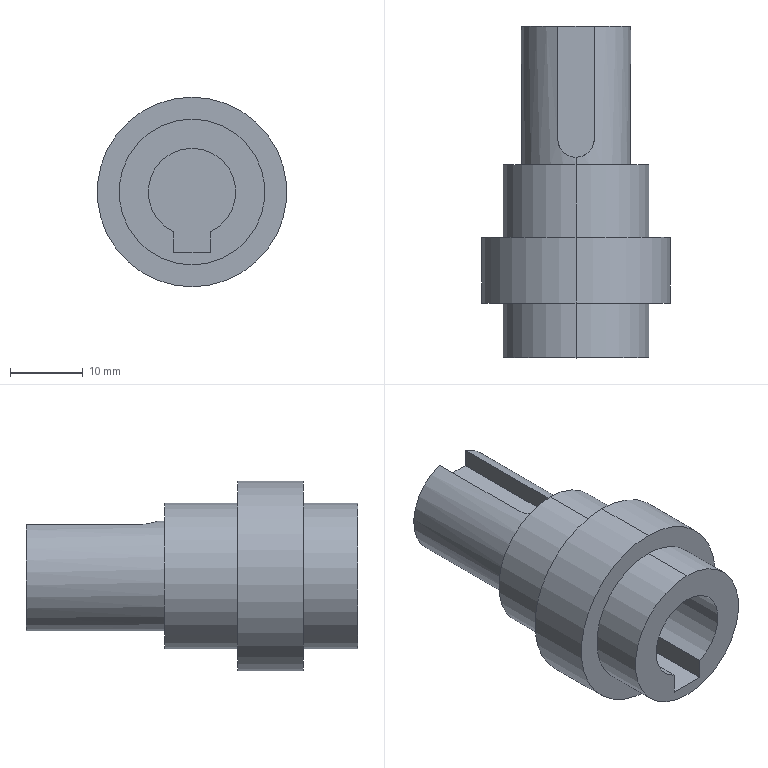Component | SolidWorks | DialAxis-1_DialAxisNo.3-1 | 1 solid | 26 faces | box 26 x 45.5 x 26 mm | volume 10013 mm3 | cylinder 12 | plane 12 | cone 2 | commonest cylinder face diameters 20 x4 3 x2 26 x2 15 x2 5 x1 12 x1
build123d program:
from build123d import *

# Parameters (mm, degrees)
CUT_EXTRUDE1_DEPTH    = 10
SKETCH3_R             = 6
CUT_EXTRUDE2_DEPTH    = 26
CUT_EXTRUDE3_DEPTH    = 26
M3_TAPPED_HOLE1_D     = 3
M3_TAPPED_HOLE1_DEPTH = 15
M3_TAPPED_HOLE1_TIP   = 0.9013


with BuildPart() as part:
    # Sketch1 → Revolve1 (revolve)
    with BuildSketch(Plane.XY, mode=Mode.PRIVATE) as revolve1_sk:
        Polygon((-29, 0), (-29, 7.5), (-10, 7.5), (-10, 10), (0, 10), (0, 13), (9, 13), (9, 10), (16.5, 10), (16.5, 9), (16.5, 0), align=None)
    revolve(revolve1_sk.sketch.rotate(Axis((-29, 0, 0), (1, 0, 0)), 90), axis=Axis((-29, 0, 0), (1, 0, 0)))

    # Sketch2 → Cut-Extrude1 (cut)
    with BuildSketch(Plane.XY.offset(4.5)):
        with BuildLine():
            Line((-29, 2.5), (-13.5, 2.5))
            ThreePointArc((-13.5, 2.5), (-11, 0), (-13.5, -2.5))
            Line((-13.5, -2.5), (-29, -2.5))
            ThreePointArc((-29, -2.5), (-31.5, 0), (-29, 2.5))
        make_face()
    extrude(amount=CUT_EXTRUDE1_DEPTH, mode=Mode.SUBTRACT)

    # Sketch3 → Cut-Extrude2 (cut)
    with BuildSketch(Plane(origin=(16.5, 0, 0), x_dir=(0, 0, -1), z_dir=(1, 0, 0))):
        Circle(SKETCH3_R)
    extrude(amount=-CUT_EXTRUDE2_DEPTH, mode=Mode.SUBTRACT)

    # Sketch4 → Cut-Extrude3 (cut)
    with BuildSketch(Plane(origin=(16.5, 0, 0), x_dir=(0, 0, -1), z_dir=(1, 0, 0))):
        with BuildLine():
            Line((8.3, 0), (6, 0))
            ThreePointArc((6, 0), (5.862, -1.279), (5.454, -2.5))
            Line((5.454, -2.5), (8.3, -2.5))
            Line((8.3, -2.5), (8.3, 0))
        make_face()
        with BuildLine():
            ThreePointArc((5.454, 2.5), (5.862, 1.279), (6, 0))
            Line((6, 0), (8.3, 0))
            Line((8.3, 0), (8.3, 2.5))
            Line((8.3, 2.5), (5.454, 2.5))
        make_face()
    extrude(amount=-CUT_EXTRUDE3_DEPTH, mode=Mode.SUBTRACT)

    # M3 Tapped Hole1
    with Locations(Plane.ZY.offset(29)):
        with Locations((0, 0)):
            Hole(M3_TAPPED_HOLE1_D / 2, depth=M3_TAPPED_HOLE1_DEPTH)
            with Locations((0, 0, -(M3_TAPPED_HOLE1_DEPTH + M3_TAPPED_HOLE1_TIP / 2))):  # 118° drill point
                Cone(0, M3_TAPPED_HOLE1_D / 2, M3_TAPPED_HOLE1_TIP, mode=Mode.SUBTRACT)


solid = part.part

# Placed as in the assembly
solid = solid.moved(Location((-96.534, 127.266, -166.507), (0, 0, -90)))
STEP:
#1=COLOUR_RGB('',0.7922,0.8196,0.9333);
#2=FILL_AREA_STYLE_COLOUR('',#1);
#3=FILL_AREA_STYLE('',(#2));
#4=SURFACE_STYLE_FILL_AREA(#3);
#5=SURFACE_SIDE_STYLE('',(#4));
#6=SURFACE_STYLE_USAGE(.BOTH.,#5);
#7=PRESENTATION_STYLE_ASSIGNMENT((#6));
#8=CARTESIAN_POINT('',(-3.801,5.562,-6.614));
#9=VERTEX_POINT('',#8);
#10=CARTESIAN_POINT('',(-3.801,5.562,-6.496));
#11=VERTEX_POINT('',#10);
#12=CARTESIAN_POINT('',(-3.801,5.562,-6.555));
#13=DIRECTION('',(0.,1.,0.));
#14=DIRECTION('',(0.,0.,1.));
#15=AXIS2_PLACEMENT_3D('',#12,#13,#14);
#16=CIRCLE('',#15,0.05906);
#17=EDGE_CURVE('',#9,#11,#16,.T.);
#18=ORIENTED_EDGE('',*,*,#17,.F.);
#19=CARTESIAN_POINT('',(-3.801,6.152,-6.614));
#20=VERTEX_POINT('',#19);
#21=CARTESIAN_POINT('',(-3.801,6.152,-6.614));
#22=DIRECTION('',(0.,1.,0.));
#23=VECTOR('',#22,39.37);
#24=LINE('',#21,#23);
#25=EDGE_CURVE('',#9,#20,#24,.T.);
#26=ORIENTED_EDGE('',*,*,#25,.T.);
#27=CARTESIAN_POINT('',(-3.801,6.152,-6.496));
#28=VERTEX_POINT('',#27);
#29=CARTESIAN_POINT('',(-3.801,6.152,-6.555));
#30=DIRECTION('',(0.,1.,0.));
#31=DIRECTION('',(0.,0.,1.));
#32=AXIS2_PLACEMENT_3D('',#29,#30,#31);
#33=CIRCLE('',#32,0.05906);
#34=EDGE_CURVE('',#20,#28,#33,.T.);
#35=ORIENTED_EDGE('',*,*,#34,.T.);
#36=CARTESIAN_POINT('',(-3.801,6.152,-6.496));
#37=DIRECTION('',(0.,1.,0.));
#38=VECTOR('',#37,39.37);
#39=LINE('',#36,#38);
#40=EDGE_CURVE('',#11,#28,#39,.T.);
#41=ORIENTED_EDGE('',*,*,#40,.F.);
#42=EDGE_LOOP('',(#18,#26,#35,#41));
#43=FACE_OUTER_BOUND('',#42,.T.);
#44=CARTESIAN_POINT('',(-3.801,6.152,-6.555));
#45=DIRECTION('',(0.,1.,0.));
#46=DIRECTION('',(0.,0.,1.));
#47=AXIS2_PLACEMENT_3D('',#44,#45,#46);
#48=CYLINDRICAL_SURFACE('',#47,0.05906);
#49=ADVANCED_FACE('',(#43),#48,.F.);
#50=CARTESIAN_POINT('',(-3.801,5.526,-6.555));
#51=VERTEX_POINT('',#50);
#52=CARTESIAN_POINT('',(-3.801,5.562,-6.496));
#53=DIRECTION('',(0.,0.515,0.8572));
#54=VECTOR('',#53,39.37);
#55=LINE('',#52,#54);
#56=EDGE_CURVE('',#51,#11,#55,.T.);
#57=ORIENTED_EDGE('',*,*,#56,.F.);
#58=CARTESIAN_POINT('',(-3.801,5.562,-6.614));
#59=DIRECTION('',(-0.,0.515,-0.8572));
#60=VECTOR('',#59,39.37);
#61=LINE('',#58,#60);
#62=EDGE_CURVE('',#51,#9,#61,.T.);
#63=ORIENTED_EDGE('',*,*,#62,.T.);
#64=ORIENTED_EDGE('',*,*,#17,.T.);
#65=EDGE_LOOP('',(#57,#63,#64));
#66=FACE_OUTER_BOUND('',#65,.T.);
#67=CARTESIAN_POINT('',(-3.801,5.562,-6.555));
#68=DIRECTION('',(0.,1.,0.));
#69=DIRECTION('',(0.,0.,1.));
#70=AXIS2_PLACEMENT_3D('',#67,#68,#69);
#71=CONICAL_SURFACE('',#70,0.05906,1.03);
#72=ADVANCED_FACE('',(#66),#71,.F.);
#73=CARTESIAN_POINT('',(-3.801,4.361,-6.162));
#74=VERTEX_POINT('',#73);
#75=CARTESIAN_POINT('',(-3.801,4.361,-6.949));
#76=VERTEX_POINT('',#75);
#77=CARTESIAN_POINT('',(-3.801,4.361,-6.555));
#78=DIRECTION('',(0.,1.,0.));
#79=DIRECTION('',(0.,0.,1.));
#80=AXIS2_PLACEMENT_3D('',#77,#78,#79);
#81=CIRCLE('',#80,0.3937);
#82=EDGE_CURVE('',#74,#76,#81,.T.);
#83=ORIENTED_EDGE('',*,*,#82,.T.);
#84=CARTESIAN_POINT('',(-3.801,4.656,-6.949));
#85=VERTEX_POINT('',#84);
#86=CARTESIAN_POINT('',(-3.801,6.152,-6.949));
#87=DIRECTION('',(0.,1.,0.));
#88=VECTOR('',#87,39.37);
#89=LINE('',#86,#88);
#90=EDGE_CURVE('',#76,#85,#89,.T.);
#91=ORIENTED_EDGE('',*,*,#90,.T.);
#92=CARTESIAN_POINT('',(-3.801,4.656,-6.162));
#93=VERTEX_POINT('',#92);
#94=CARTESIAN_POINT('',(-3.801,4.656,-6.555));
#95=DIRECTION('',(0.,1.,0.));
#96=DIRECTION('',(0.,0.,1.));
#97=AXIS2_PLACEMENT_3D('',#94,#95,#96);
#98=CIRCLE('',#97,0.3937);
#99=EDGE_CURVE('',#93,#85,#98,.T.);
#100=ORIENTED_EDGE('',*,*,#99,.F.);
#101=CARTESIAN_POINT('',(-3.801,6.152,-6.162));
#102=DIRECTION('',(0.,1.,0.));
#103=VECTOR('',#102,39.37);
#104=LINE('',#101,#103);
#105=EDGE_CURVE('',#74,#93,#104,.T.);
#106=ORIENTED_EDGE('',*,*,#105,.F.);
#107=EDGE_LOOP('',(#83,#91,#100,#106));
#108=FACE_OUTER_BOUND('',#107,.T.);
#109=CARTESIAN_POINT('',(-3.801,6.152,-6.555));
#110=DIRECTION('',(0.,1.,0.));
#111=DIRECTION('',(0.,0.,1.));
#112=AXIS2_PLACEMENT_3D('',#109,#110,#111);
#113=CYLINDRICAL_SURFACE('',#112,0.3937);
#114=ADVANCED_FACE('',(#108),#113,.T.);
#115=CARTESIAN_POINT('',(-3.801,4.656,-6.044));
#116=VERTEX_POINT('',#115);
#117=CARTESIAN_POINT('',(-3.801,4.656,-7.067));
#118=VERTEX_POINT('',#117);
#119=CARTESIAN_POINT('',(-3.801,4.656,-6.555));
#120=DIRECTION('',(0.,1.,0.));
#121=DIRECTION('',(0.,0.,1.));
#122=AXIS2_PLACEMENT_3D('',#119,#120,#121);
#123=CIRCLE('',#122,0.5118);
#124=EDGE_CURVE('',#116,#118,#123,.T.);
#125=ORIENTED_EDGE('',*,*,#124,.T.);
#126=CARTESIAN_POINT('',(-3.801,5.01,-7.067));
#127=VERTEX_POINT('',#126);
#128=CARTESIAN_POINT('',(-3.801,6.152,-7.067));
#129=DIRECTION('',(0.,1.,0.));
#130=VECTOR('',#129,39.37);
#131=LINE('',#128,#130);
#132=EDGE_CURVE('',#118,#127,#131,.T.);
#133=ORIENTED_EDGE('',*,*,#132,.T.);
#134=CARTESIAN_POINT('',(-3.801,5.01,-6.044));
#135=VERTEX_POINT('',#134);
#136=CARTESIAN_POINT('',(-3.801,5.01,-6.555));
#137=DIRECTION('',(0.,1.,0.));
#138=DIRECTION('',(0.,0.,1.));
#139=AXIS2_PLACEMENT_3D('',#136,#137,#138);
#140=CIRCLE('',#139,0.5118);
#141=EDGE_CURVE('',#135,#127,#140,.T.);
#142=ORIENTED_EDGE('',*,*,#141,.F.);
#143=CARTESIAN_POINT('',(-3.801,6.152,-6.044));
#144=DIRECTION('',(0.,1.,0.));
#145=VECTOR('',#144,39.37);
#146=LINE('',#143,#145);
#147=EDGE_CURVE('',#116,#135,#146,.T.);
#148=ORIENTED_EDGE('',*,*,#147,.F.);
#149=EDGE_LOOP('',(#125,#133,#142,#148));
#150=FACE_OUTER_BOUND('',#149,.T.);
#151=CARTESIAN_POINT('',(-3.801,6.152,-6.555));
#152=DIRECTION('',(0.,1.,0.));
#153=DIRECTION('',(0.,0.,1.));
#154=AXIS2_PLACEMENT_3D('',#151,#152,#153);
#155=CYLINDRICAL_SURFACE('',#154,0.5118);
#156=ADVANCED_FACE('',(#150),#155,.T.);
#157=CARTESIAN_POINT('',(-3.801,5.01,-6.162));
#158=VERTEX_POINT('',#157);
#159=CARTESIAN_POINT('',(-3.801,5.01,-6.949));
#160=VERTEX_POINT('',#159);
#161=CARTESIAN_POINT('',(-3.801,5.01,-6.555));
#162=DIRECTION('',(0.,1.,0.));
#163=DIRECTION('',(0.,0.,1.));
#164=AXIS2_PLACEMENT_3D('',#161,#162,#163);
#165=CIRCLE('',#164,0.3937);
#166=EDGE_CURVE('',#158,#160,#165,.T.);
#167=ORIENTED_EDGE('',*,*,#166,.T.);
#168=CARTESIAN_POINT('',(-3.801,5.404,-6.949));
#169=VERTEX_POINT('',#168);
#170=CARTESIAN_POINT('',(-3.801,6.152,-6.949));
#171=DIRECTION('',(0.,1.,0.));
#172=VECTOR('',#171,39.37);
#173=LINE('',#170,#172);
#174=EDGE_CURVE('',#160,#169,#173,.T.);
#175=ORIENTED_EDGE('',*,*,#174,.T.);
#176=CARTESIAN_POINT('',(-3.801,5.404,-6.162));
#177=VERTEX_POINT('',#176);
#178=CARTESIAN_POINT('',(-3.801,5.404,-6.555));
#179=DIRECTION('',(0.,1.,0.));
#180=DIRECTION('',(0.,0.,1.));
#181=AXIS2_PLACEMENT_3D('',#178,#179,#180);
#182=CIRCLE('',#181,0.3937);
#183=EDGE_CURVE('',#177,#169,#182,.T.);
#184=ORIENTED_EDGE('',*,*,#183,.F.);
#185=CARTESIAN_POINT('',(-3.801,6.152,-6.162));
#186=DIRECTION('',(0.,1.,0.));
#187=VECTOR('',#186,39.37);
#188=LINE('',#185,#187);
#189=EDGE_CURVE('',#158,#177,#188,.T.);
#190=ORIENTED_EDGE('',*,*,#189,.F.);
#191=EDGE_LOOP('',(#167,#175,#184,#190));
#192=FACE_OUTER_BOUND('',#191,.T.);
#193=CARTESIAN_POINT('',(-3.801,6.152,-6.555));
#194=DIRECTION('',(0.,1.,0.));
#195=DIRECTION('',(0.,0.,1.));
#196=AXIS2_PLACEMENT_3D('',#193,#194,#195);
#197=CYLINDRICAL_SURFACE('',#196,0.3937);
#198=ADVANCED_FACE('',(#192),#197,.T.);
#199=CARTESIAN_POINT('',(-3.801,5.404,-6.26));
#200=VERTEX_POINT('',#199);
#201=CARTESIAN_POINT('',(-3.801,5.404,-6.851));
#202=VERTEX_POINT('',#201);
#203=CARTESIAN_POINT('',(-3.801,5.404,-6.555));
#204=DIRECTION('',(0.,1.,0.));
#205=DIRECTION('',(0.,0.,1.));
#206=AXIS2_PLACEMENT_3D('',#203,#204,#205);
#207=CIRCLE('',#206,0.2953);
#208=EDGE_CURVE('',#200,#202,#207,.T.);
#209=ORIENTED_EDGE('',*,*,#208,.T.);
#210=CARTESIAN_POINT('',(-3.801,6.152,-6.851));
#211=VERTEX_POINT('',#210);
#212=CARTESIAN_POINT('',(-3.801,6.152,-6.851));
#213=DIRECTION('',(0.,1.,0.));
#214=VECTOR('',#213,39.37);
#215=LINE('',#212,#214);
#216=EDGE_CURVE('',#202,#211,#215,.T.);
#217=ORIENTED_EDGE('',*,*,#216,.T.);
#218=CARTESIAN_POINT('',(-3.702,6.152,-6.277));
#219=VERTEX_POINT('',#218);
#220=CARTESIAN_POINT('',(-3.801,6.152,-6.555));
#221=DIRECTION('',(0.,1.,0.));
#222=DIRECTION('',(0.,0.,1.));
#223=AXIS2_PLACEMENT_3D('',#220,#221,#222);
#224=CIRCLE('',#223,0.2953);
#225=EDGE_CURVE('',#219,#211,#224,.T.);
#226=ORIENTED_EDGE('',*,*,#225,.F.);
#227=CARTESIAN_POINT('',(-3.702,5.542,-6.277));
#228=VERTEX_POINT('',#227);
#229=CARTESIAN_POINT('',(-3.702,6.152,-6.277));
#230=DIRECTION('',(0.,1.,0.));
#231=VECTOR('',#230,39.37);
#232=LINE('',#229,#231);
#233=EDGE_CURVE('',#228,#219,#232,.T.);
#234=ORIENTED_EDGE('',*,*,#233,.F.);
#235=CARTESIAN_POINT('',(-3.801,5.444,-6.26));
#236=VERTEX_POINT('',#235);
#237=CARTESIAN_POINT('',(-3.801,5.444,-6.26));
#238=CARTESIAN_POINT('',(-3.794,5.444,-6.26));
#239=CARTESIAN_POINT('',(-3.788,5.444,-6.26));
#240=CARTESIAN_POINT('',(-3.775,5.447,-6.261));
#241=CARTESIAN_POINT('',(-3.769,5.449,-6.262));
#242=CARTESIAN_POINT('',(-3.757,5.454,-6.263));
#243=CARTESIAN_POINT('',(-3.751,5.457,-6.264));
#244=CARTESIAN_POINT('',(-3.74,5.464,-6.266));
#245=CARTESIAN_POINT('',(-3.735,5.468,-6.267));
#246=CARTESIAN_POINT('',(-3.726,5.477,-6.27));
#247=CARTESIAN_POINT('',(-3.722,5.482,-6.271));
#248=CARTESIAN_POINT('',(-3.715,5.492,-6.273));
#249=CARTESIAN_POINT('',(-3.712,5.498,-6.274));
#250=CARTESIAN_POINT('',(-3.707,5.51,-6.275));
#251=CARTESIAN_POINT('',(-3.705,5.516,-6.276));
#252=CARTESIAN_POINT('',(-3.703,5.529,-6.277));
#253=CARTESIAN_POINT('',(-3.702,5.535,-6.277));
#254=CARTESIAN_POINT('',(-3.702,5.542,-6.277));
#255=B_SPLINE_CURVE_WITH_KNOTS('',3,(#237,#238,#239,#240,#241,#242,#243,#244,#245,#246,#247,#248,#249,#250,#251,#252,#253,#254),.UNSPECIFIED.,.F.,.F.,(4,2,2,2,2,2,2,2,4),(0.003937,0.004429,0.004921,0.005412,0.005904,0.006395,0.006887,0.007378,0.00787),.UNSPECIFIED.);
#256=EDGE_CURVE('',#236,#228,#255,.T.);
#257=ORIENTED_EDGE('',*,*,#256,.F.);
#258=CARTESIAN_POINT('',(-3.801,6.152,-6.26));
#259=DIRECTION('',(0.,1.,0.));
#260=VECTOR('',#259,39.37);
#261=LINE('',#258,#260);
#262=EDGE_CURVE('',#200,#236,#261,.T.);
#263=ORIENTED_EDGE('',*,*,#262,.F.);
#264=EDGE_LOOP('',(#209,#217,#226,#234,#257,#263));
#265=FACE_OUTER_BOUND('',#264,.T.);
#266=CARTESIAN_POINT('',(-3.801,6.152,-6.555));
#267=DIRECTION('',(0.,1.,0.));
#268=DIRECTION('',(0.,0.,1.));
#269=AXIS2_PLACEMENT_3D('',#266,#267,#268);
#270=CYLINDRICAL_SURFACE('',#269,0.2953);
#271=ADVANCED_FACE('',(#265),#270,.T.);
#272=CARTESIAN_POINT('',(-3.801,6.152,-6.555));
#273=DIRECTION('',(0.,1.,0.));
#274=DIRECTION('',(0.,0.,1.));
#275=AXIS2_PLACEMENT_3D('',#272,#273,#274);
#276=CIRCLE('',#275,0.05906);
#277=EDGE_CURVE('',#28,#20,#276,.T.);
#278=ORIENTED_EDGE('',*,*,#277,.F.);
#279=ORIENTED_EDGE('',*,*,#34,.F.);
#280=EDGE_LOOP('',(#278,#279));
#281=FACE_BOUND('',#280,.T.);
#282=CARTESIAN_POINT('',(-3.899,6.152,-6.277));
#283=VERTEX_POINT('',#282);
#284=CARTESIAN_POINT('',(-3.899,6.152,-6.378));
#285=VERTEX_POINT('',#284);
#286=CARTESIAN_POINT('',(-3.899,6.152,-5.985));
#287=DIRECTION('',(-0.,0.,-1.));
#288=VECTOR('',#287,39.37);
#289=LINE('',#286,#288);
#290=EDGE_CURVE('',#283,#285,#289,.T.);
#291=ORIENTED_EDGE('',*,*,#290,.T.);
#292=CARTESIAN_POINT('',(-3.702,6.152,-6.378));
#293=VERTEX_POINT('',#292);
#294=CARTESIAN_POINT('',(-3.801,6.152,-6.378));
#295=DIRECTION('',(-1.,0.,0.));
#296=VECTOR('',#295,39.37);
#297=LINE('',#294,#296);
#298=EDGE_CURVE('',#293,#285,#297,.T.);
#299=ORIENTED_EDGE('',*,*,#298,.F.);
#300=CARTESIAN_POINT('',(-3.702,6.152,-5.985));
#301=DIRECTION('',(-0.,0.,-1.));
#302=VECTOR('',#301,39.37);
#303=LINE('',#300,#302);
#304=EDGE_CURVE('',#219,#293,#303,.T.);
#305=ORIENTED_EDGE('',*,*,#304,.F.);
#306=ORIENTED_EDGE('',*,*,#225,.T.);
#307=CARTESIAN_POINT('',(-3.801,6.152,-6.555));
#308=DIRECTION('',(0.,1.,0.));
#309=DIRECTION('',(0.,0.,1.));
#310=AXIS2_PLACEMENT_3D('',#307,#308,#309);
#311=CIRCLE('',#310,0.2953);
#312=EDGE_CURVE('',#211,#283,#311,.T.);
#313=ORIENTED_EDGE('',*,*,#312,.T.);
#314=EDGE_LOOP('',(#291,#299,#305,#306,#313));
#315=FACE_OUTER_BOUND('',#314,.T.);
#316=CARTESIAN_POINT('',(-3.801,6.152,-6.555));
#317=DIRECTION('',(0.,-1.,0.));
#318=DIRECTION('',(-0.,0.,-1.));
#319=AXIS2_PLACEMENT_3D('',#316,#317,#318);
#320=PLANE('',#319);
#321=ADVANCED_FACE('',(#281,#315),#320,.F.);
#322=ORIENTED_EDGE('',*,*,#216,.F.);
#323=CARTESIAN_POINT('',(-3.801,5.404,-6.555));
#324=DIRECTION('',(0.,1.,0.));
#325=DIRECTION('',(0.,0.,1.));
#326=AXIS2_PLACEMENT_3D('',#323,#324,#325);
#327=CIRCLE('',#326,0.2953);
#328=EDGE_CURVE('',#202,#200,#327,.T.);
#329=ORIENTED_EDGE('',*,*,#328,.T.);
#330=ORIENTED_EDGE('',*,*,#262,.T.);
#331=CARTESIAN_POINT('',(-3.899,5.542,-6.277));
#332=VERTEX_POINT('',#331);
#333=CARTESIAN_POINT('',(-3.899,5.542,-6.277));
#334=CARTESIAN_POINT('',(-3.899,5.535,-6.277));
#335=CARTESIAN_POINT('',(-3.898,5.529,-6.277));
#336=CARTESIAN_POINT('',(-3.896,5.516,-6.276));
#337=CARTESIAN_POINT('',(-3.894,5.51,-6.275));
#338=CARTESIAN_POINT('',(-3.889,5.498,-6.274));
#339=CARTESIAN_POINT('',(-3.886,5.493,-6.273));
#340=CARTESIAN_POINT('',(-3.879,5.482,-6.271));
#341=CARTESIAN_POINT('',(-3.875,5.477,-6.27));
#342=CARTESIAN_POINT('',(-3.861,5.463,-6.266));
#343=CARTESIAN_POINT('',(-3.85,5.456,-6.264));
#344=CARTESIAN_POINT('',(-3.832,5.449,-6.262));
#345=CARTESIAN_POINT('',(-3.826,5.447,-6.261));
#346=CARTESIAN_POINT('',(-3.813,5.444,-6.26));
#347=CARTESIAN_POINT('',(-3.807,5.444,-6.26));
#348=CARTESIAN_POINT('',(-3.801,5.444,-6.26));
#349=B_SPLINE_CURVE_WITH_KNOTS('',3,(#333,#334,#335,#336,#337,#338,#339,#340,#341,#342,#343,#344,#345,#346,#347,#348),.UNSPECIFIED.,.F.,.F.,(4,2,2,2,2,2,2,4),(0.,0.0004922,0.0009844,0.001477,0.001969,0.002953,0.003445,0.003937),.UNSPECIFIED.);
#350=EDGE_CURVE('',#332,#236,#349,.T.);
#351=ORIENTED_EDGE('',*,*,#350,.F.);
#352=CARTESIAN_POINT('',(-3.899,6.152,-6.277));
#353=DIRECTION('',(0.,-1.,0.));
#354=VECTOR('',#353,39.37);
#355=LINE('',#352,#354);
#356=EDGE_CURVE('',#283,#332,#355,.T.);
#357=ORIENTED_EDGE('',*,*,#356,.F.);
#358=ORIENTED_EDGE('',*,*,#312,.F.);
#359=EDGE_LOOP('',(#322,#329,#330,#351,#357,#358));
#360=FACE_OUTER_BOUND('',#359,.T.);
#361=CARTESIAN_POINT('',(-3.801,6.152,-6.555));
#362=DIRECTION('',(0.,1.,0.));
#363=DIRECTION('',(0.,0.,1.));
#364=AXIS2_PLACEMENT_3D('',#361,#362,#363);
#365=CYLINDRICAL_SURFACE('',#364,0.2953);
#366=ADVANCED_FACE('',(#360),#365,.T.);
#367=ORIENTED_EDGE('',*,*,#208,.F.);
#368=ORIENTED_EDGE('',*,*,#328,.F.);
#369=EDGE_LOOP('',(#367,#368));
#370=FACE_BOUND('',#369,.T.);
#371=ORIENTED_EDGE('',*,*,#183,.T.);
#372=CARTESIAN_POINT('',(-3.801,5.404,-6.555));
#373=DIRECTION('',(0.,1.,0.));
#374=DIRECTION('',(0.,0.,1.));
#375=AXIS2_PLACEMENT_3D('',#372,#373,#374);
#376=CIRCLE('',#375,0.3937);
#377=EDGE_CURVE('',#169,#177,#376,.T.);
#378=ORIENTED_EDGE('',*,*,#377,.T.);
#379=EDGE_LOOP('',(#371,#378));
#380=FACE_OUTER_BOUND('',#379,.T.);
#381=CARTESIAN_POINT('',(-3.505,5.404,-6.555));
#382=DIRECTION('',(0.,-1.,0.));
#383=DIRECTION('',(-0.,0.,-1.));
#384=AXIS2_PLACEMENT_3D('',#381,#382,#383);
#385=PLANE('',#384);
#386=ADVANCED_FACE('',(#370,#380),#385,.F.);
#387=ORIENTED_EDGE('',*,*,#174,.F.);
#388=CARTESIAN_POINT('',(-3.801,5.01,-6.555));
#389=DIRECTION('',(0.,1.,0.));
#390=DIRECTION('',(0.,0.,1.));
#391=AXIS2_PLACEMENT_3D('',#388,#389,#390);
#392=CIRCLE('',#391,0.3937);
#393=EDGE_CURVE('',#160,#158,#392,.T.);
#394=ORIENTED_EDGE('',*,*,#393,.T.);
#395=ORIENTED_EDGE('',*,*,#189,.T.);
#396=ORIENTED_EDGE('',*,*,#377,.F.);
#397=EDGE_LOOP('',(#387,#394,#395,#396));
#398=FACE_OUTER_BOUND('',#397,.T.);
#399=CARTESIAN_POINT('',(-3.801,6.152,-6.555));
#400=DIRECTION('',(0.,1.,0.));
#401=DIRECTION('',(0.,0.,1.));
#402=AXIS2_PLACEMENT_3D('',#399,#400,#401);
#403=CYLINDRICAL_SURFACE('',#402,0.3937);
#404=ADVANCED_FACE('',(#398),#403,.T.);
#405=ORIENTED_EDGE('',*,*,#166,.F.);
#406=ORIENTED_EDGE('',*,*,#393,.F.);
#407=EDGE_LOOP('',(#405,#406));
#408=FACE_BOUND('',#407,.T.);
#409=ORIENTED_EDGE('',*,*,#141,.T.);
#410=CARTESIAN_POINT('',(-3.801,5.01,-6.555));
#411=DIRECTION('',(0.,1.,0.));
#412=DIRECTION('',(0.,0.,1.));
#413=AXIS2_PLACEMENT_3D('',#410,#411,#412);
#414=CIRCLE('',#413,0.5118);
#415=EDGE_CURVE('',#127,#135,#414,.T.);
#416=ORIENTED_EDGE('',*,*,#415,.T.);
#417=EDGE_LOOP('',(#409,#416));
#418=FACE_OUTER_BOUND('',#417,.T.);
#419=CARTESIAN_POINT('',(-3.407,5.01,-6.555));
#420=DIRECTION('',(0.,-1.,0.));
#421=DIRECTION('',(-0.,0.,-1.));
#422=AXIS2_PLACEMENT_3D('',#419,#420,#421);
#423=PLANE('',#422);
#424=ADVANCED_FACE('',(#408,#418),#423,.F.);
#425=ORIENTED_EDGE('',*,*,#132,.F.);
#426=CARTESIAN_POINT('',(-3.801,4.656,-6.555));
#427=DIRECTION('',(0.,1.,0.));
#428=DIRECTION('',(0.,0.,1.));
#429=AXIS2_PLACEMENT_3D('',#426,#427,#428);
#430=CIRCLE('',#429,0.5118);
#431=EDGE_CURVE('',#118,#116,#430,.T.);
#432=ORIENTED_EDGE('',*,*,#431,.T.);
#433=ORIENTED_EDGE('',*,*,#147,.T.);
#434=ORIENTED_EDGE('',*,*,#415,.F.);
#435=EDGE_LOOP('',(#425,#432,#433,#434));
#436=FACE_OUTER_BOUND('',#435,.T.);
#437=CARTESIAN_POINT('',(-3.801,6.152,-6.555));
#438=DIRECTION('',(0.,1.,0.));
#439=DIRECTION('',(0.,0.,1.));
#440=AXIS2_PLACEMENT_3D('',#437,#438,#439);
#441=CYLINDRICAL_SURFACE('',#440,0.5118);
#442=ADVANCED_FACE('',(#436),#441,.T.);
#443=ORIENTED_EDGE('',*,*,#124,.F.);
#444=ORIENTED_EDGE('',*,*,#431,.F.);
#445=EDGE_LOOP('',(#443,#444));
#446=FACE_OUTER_BOUND('',#445,.T.);
#447=ORIENTED_EDGE('',*,*,#99,.T.);
#448=CARTESIAN_POINT('',(-3.801,4.656,-6.555));
#449=DIRECTION('',(0.,1.,0.));
#450=DIRECTION('',(0.,0.,1.));
#451=AXIS2_PLACEMENT_3D('',#448,#449,#450);
#452=CIRCLE('',#451,0.3937);
#453=EDGE_CURVE('',#85,#93,#452,.T.);
#454=ORIENTED_EDGE('',*,*,#453,.T.);
#455=EDGE_LOOP('',(#447,#454));
#456=FACE_BOUND('',#455,.T.);
#457=CARTESIAN_POINT('',(-3.289,4.656,-6.555));
#458=DIRECTION('',(0.,1.,0.));
#459=DIRECTION('',(0.,0.,1.));
#460=AXIS2_PLACEMENT_3D('',#457,#458,#459);
#461=PLANE('',#460);
#462=ADVANCED_FACE('',(#446,#456),#461,.F.);
#463=ORIENTED_EDGE('',*,*,#90,.F.);
#464=CARTESIAN_POINT('',(-3.801,4.361,-6.555));
#465=DIRECTION('',(0.,1.,0.));
#466=DIRECTION('',(0.,0.,1.));
#467=AXIS2_PLACEMENT_3D('',#464,#465,#466);
#468=CIRCLE('',#467,0.3937);
#469=EDGE_CURVE('',#76,#74,#468,.T.);
#470=ORIENTED_EDGE('',*,*,#469,.T.);
#471=ORIENTED_EDGE('',*,*,#105,.T.);
#472=ORIENTED_EDGE('',*,*,#453,.F.);
#473=EDGE_LOOP('',(#463,#470,#471,#472));
#474=FACE_OUTER_BOUND('',#473,.T.);
#475=CARTESIAN_POINT('',(-3.801,6.152,-6.555));
#476=DIRECTION('',(0.,1.,0.));
#477=DIRECTION('',(0.,0.,1.));
#478=AXIS2_PLACEMENT_3D('',#475,#476,#477);
#479=CYLINDRICAL_SURFACE('',#478,0.3937);
#480=ADVANCED_FACE('',(#474),#479,.T.);
#481=CARTESIAN_POINT('',(-3.702,4.361,-6.882));
#482=VERTEX_POINT('',#481);
#483=CARTESIAN_POINT('',(-3.899,4.361,-6.882));
#484=VERTEX_POINT('',#483);
#485=CARTESIAN_POINT('',(-3.801,4.361,-6.882));
#486=DIRECTION('',(-1.,0.,0.));
#487=VECTOR('',#486,39.37);
#488=LINE('',#485,#487);
#489=EDGE_CURVE('',#482,#484,#488,.T.);
#490=ORIENTED_EDGE('',*,*,#489,.T.);
#491=CARTESIAN_POINT('',(-3.899,4.361,-6.77));
#492=VERTEX_POINT('',#491);
#493=CARTESIAN_POINT('',(-3.899,4.361,-6.555));
#494=DIRECTION('',(-0.,0.,-1.));
#495=VECTOR('',#494,39.37);
#496=LINE('',#493,#495);
#497=EDGE_CURVE('',#492,#484,#496,.T.);
#498=ORIENTED_EDGE('',*,*,#497,.F.);
#499=CARTESIAN_POINT('',(-3.702,4.361,-6.77));
#500=VERTEX_POINT('',#499);
#501=CARTESIAN_POINT('',(-3.801,4.361,-6.555));
#502=DIRECTION('',(0.,-1.,0.));
#503=DIRECTION('',(0.,0.,-1.));
#504=AXIS2_PLACEMENT_3D('',#501,#502,#503);
#505=CIRCLE('',#504,0.2362);
#506=EDGE_CURVE('',#500,#492,#505,.T.);
#507=ORIENTED_EDGE('',*,*,#506,.F.);
#508=CARTESIAN_POINT('',(-3.702,4.361,-6.555));
#509=DIRECTION('',(-0.,0.,-1.));
#510=VECTOR('',#509,39.37);
#511=LINE('',#508,#510);
#512=EDGE_CURVE('',#500,#482,#511,.T.);
#513=ORIENTED_EDGE('',*,*,#512,.T.);
#514=EDGE_LOOP('',(#490,#498,#507,#513));
#515=FACE_BOUND('',#514,.T.);
#516=ORIENTED_EDGE('',*,*,#82,.F.);
#517=ORIENTED_EDGE('',*,*,#469,.F.);
#518=EDGE_LOOP('',(#516,#517));
#519=FACE_OUTER_BOUND('',#518,.T.);
#520=CARTESIAN_POINT('',(-3.446,4.361,-6.555));
#521=DIRECTION('',(0.,1.,0.));
#522=DIRECTION('',(0.,0.,1.));
#523=AXIS2_PLACEMENT_3D('',#520,#521,#522);
#524=PLANE('',#523);
#525=ADVANCED_FACE('',(#515,#519),#524,.F.);
#526=ORIENTED_EDGE('',*,*,#298,.T.);
#527=CARTESIAN_POINT('',(-3.899,5.542,-6.378));
#528=VERTEX_POINT('',#527);
#529=CARTESIAN_POINT('',(-3.899,6.152,-6.378));
#530=DIRECTION('',(0.,-1.,0.));
#531=VECTOR('',#530,39.37);
#532=LINE('',#529,#531);
#533=EDGE_CURVE('',#285,#528,#532,.T.);
#534=ORIENTED_EDGE('',*,*,#533,.T.);
#535=CARTESIAN_POINT('',(-3.702,5.542,-6.378));
#536=VERTEX_POINT('',#535);
#537=CARTESIAN_POINT('',(-3.801,5.542,-6.378));
#538=DIRECTION('',(0.,0.,1.));
#539=DIRECTION('',(0.,-1.,0.));
#540=AXIS2_PLACEMENT_3D('',#537,#538,#539);
#541=CIRCLE('',#540,0.09843);
#542=EDGE_CURVE('',#528,#536,#541,.T.);
#543=ORIENTED_EDGE('',*,*,#542,.T.);
#544=CARTESIAN_POINT('',(-3.702,6.152,-6.378));
#545=DIRECTION('',(0.,1.,0.));
#546=VECTOR('',#545,39.37);
#547=LINE('',#544,#546);
#548=EDGE_CURVE('',#536,#293,#547,.T.);
#549=ORIENTED_EDGE('',*,*,#548,.T.);
#550=EDGE_LOOP('',(#526,#534,#543,#549));
#551=FACE_OUTER_BOUND('',#550,.T.);
#552=CARTESIAN_POINT('',(-3.801,6.152,-6.378));
#553=DIRECTION('',(0.,0.,1.));
#554=DIRECTION('',(0.,-1.,0.));
#555=AXIS2_PLACEMENT_3D('',#552,#553,#554);
#556=PLANE('',#555);
#557=ADVANCED_FACE('',(#551),#556,.T.);
#558=ORIENTED_EDGE('',*,*,#356,.T.);
#559=CARTESIAN_POINT('',(-3.899,5.542,-5.985));
#560=DIRECTION('',(-0.,0.,-1.));
#561=VECTOR('',#560,39.37);
#562=LINE('',#559,#561);
#563=EDGE_CURVE('',#332,#528,#562,.T.);
#564=ORIENTED_EDGE('',*,*,#563,.T.);
#565=ORIENTED_EDGE('',*,*,#533,.F.);
#566=ORIENTED_EDGE('',*,*,#290,.F.);
#567=EDGE_LOOP('',(#558,#564,#565,#566));
#568=FACE_OUTER_BOUND('',#567,.T.);
#569=CARTESIAN_POINT('',(-3.899,6.152,-5.985));
#570=DIRECTION('',(1.,0.,-0.));
#571=DIRECTION('',(0.,0.,1.));
#572=AXIS2_PLACEMENT_3D('',#569,#570,#571);
#573=PLANE('',#572);
#574=ADVANCED_FACE('',(#568),#573,.T.);
#575=ORIENTED_EDGE('',*,*,#350,.T.);
#576=ORIENTED_EDGE('',*,*,#256,.T.);
#577=CARTESIAN_POINT('',(-3.702,5.542,-5.985));
#578=DIRECTION('',(-0.,0.,-1.));
#579=VECTOR('',#578,39.37);
#580=LINE('',#577,#579);
#581=EDGE_CURVE('',#228,#536,#580,.T.);
#582=ORIENTED_EDGE('',*,*,#581,.T.);
#583=ORIENTED_EDGE('',*,*,#542,.F.);
#584=ORIENTED_EDGE('',*,*,#563,.F.);
#585=EDGE_LOOP('',(#575,#576,#582,#583,#584));
#586=FACE_OUTER_BOUND('',#585,.T.);
#587=CARTESIAN_POINT('',(-3.801,5.542,-5.985));
#588=DIRECTION('',(-0.,0.,-1.));
#589=DIRECTION('',(0.,1.,0.));
#590=AXIS2_PLACEMENT_3D('',#587,#588,#589);
#591=CYLINDRICAL_SURFACE('',#590,0.09843);
#592=ADVANCED_FACE('',(#586),#591,.F.);
#593=ORIENTED_EDGE('',*,*,#233,.T.);
#594=ORIENTED_EDGE('',*,*,#304,.T.);
#595=ORIENTED_EDGE('',*,*,#548,.F.);
#596=ORIENTED_EDGE('',*,*,#581,.F.);
#597=EDGE_LOOP('',(#593,#594,#595,#596));
#598=FACE_OUTER_BOUND('',#597,.T.);
#599=CARTESIAN_POINT('',(-3.702,6.152,-5.985));
#600=DIRECTION('',(-1.,0.,0.));
#601=DIRECTION('',(-0.,0.,-1.));
#602=AXIS2_PLACEMENT_3D('',#599,#600,#601);
#603=PLANE('',#602);
#604=ADVANCED_FACE('',(#598),#603,.T.);
#605=ORIENTED_EDGE('',*,*,#506,.T.);
#606=CARTESIAN_POINT('',(-3.899,5.384,-6.77));
#607=VERTEX_POINT('',#606);
#608=CARTESIAN_POINT('',(-3.899,5.384,-6.77));
#609=DIRECTION('',(0.,-1.,0.));
#610=VECTOR('',#609,39.37);
#611=LINE('',#608,#610);
#612=EDGE_CURVE('',#607,#492,#611,.T.);
#613=ORIENTED_EDGE('',*,*,#612,.F.);
#614=CARTESIAN_POINT('',(-3.702,5.384,-6.77));
#615=VERTEX_POINT('',#614);
#616=CARTESIAN_POINT('',(-3.801,5.384,-6.555));
#617=DIRECTION('',(0.,-1.,0.));
#618=DIRECTION('',(0.,0.,-1.));
#619=AXIS2_PLACEMENT_3D('',#616,#617,#618);
#620=CIRCLE('',#619,0.2362);
#621=EDGE_CURVE('',#615,#607,#620,.T.);
#622=ORIENTED_EDGE('',*,*,#621,.F.);
#623=CARTESIAN_POINT('',(-3.702,5.384,-6.77));
#624=DIRECTION('',(0.,-1.,0.));
#625=VECTOR('',#624,39.37);
#626=LINE('',#623,#625);
#627=EDGE_CURVE('',#615,#500,#626,.T.);
#628=ORIENTED_EDGE('',*,*,#627,.T.);
#629=EDGE_LOOP('',(#605,#613,#622,#628));
#630=FACE_OUTER_BOUND('',#629,.T.);
#631=CARTESIAN_POINT('',(-3.801,5.384,-6.555));
#632=DIRECTION('',(0.,-1.,0.));
#633=DIRECTION('',(0.,0.,-1.));
#634=AXIS2_PLACEMENT_3D('',#631,#632,#633);
#635=CYLINDRICAL_SURFACE('',#634,0.2362);
#636=ADVANCED_FACE('',(#630),#635,.F.);
#637=ORIENTED_EDGE('',*,*,#621,.T.);
#638=CARTESIAN_POINT('',(-3.899,5.384,-6.882));
#639=VERTEX_POINT('',#638);
#640=CARTESIAN_POINT('',(-3.899,5.384,-6.555));
#641=DIRECTION('',(-0.,0.,-1.));
#642=VECTOR('',#641,39.37);
#643=LINE('',#640,#642);
#644=EDGE_CURVE('',#607,#639,#643,.T.);
#645=ORIENTED_EDGE('',*,*,#644,.T.);
#646=CARTESIAN_POINT('',(-3.702,5.384,-6.882));
#647=VERTEX_POINT('',#646);
#648=CARTESIAN_POINT('',(-3.801,5.384,-6.882));
#649=DIRECTION('',(-1.,0.,0.));
#650=VECTOR('',#649,39.37);
#651=LINE('',#648,#650);
#652=EDGE_CURVE('',#647,#639,#651,.T.);
#653=ORIENTED_EDGE('',*,*,#652,.F.);
#654=CARTESIAN_POINT('',(-3.702,5.384,-6.555));
#655=DIRECTION('',(-0.,0.,-1.));
#656=VECTOR('',#655,39.37);
#657=LINE('',#654,#656);
#658=EDGE_CURVE('',#615,#647,#657,.T.);
#659=ORIENTED_EDGE('',*,*,#658,.F.);
#660=EDGE_LOOP('',(#637,#645,#653,#659));
#661=FACE_OUTER_BOUND('',#660,.T.);
#662=CARTESIAN_POINT('',(-3.801,5.384,-6.555));
#663=DIRECTION('',(0.,-1.,0.));
#664=DIRECTION('',(-0.,0.,-1.));
#665=AXIS2_PLACEMENT_3D('',#662,#663,#664);
#666=PLANE('',#665);
#667=ADVANCED_FACE('',(#661),#666,.T.);
#668=ORIENTED_EDGE('',*,*,#489,.F.);
#669=CARTESIAN_POINT('',(-3.702,5.384,-6.882));
#670=DIRECTION('',(0.,-1.,0.));
#671=VECTOR('',#670,39.37);
#672=LINE('',#669,#671);
#673=EDGE_CURVE('',#647,#482,#672,.T.);
#674=ORIENTED_EDGE('',*,*,#673,.F.);
#675=ORIENTED_EDGE('',*,*,#652,.T.);
#676=CARTESIAN_POINT('',(-3.899,5.384,-6.882));
#677=DIRECTION('',(0.,-1.,0.));
#678=VECTOR('',#677,39.37);
#679=LINE('',#676,#678);
#680=EDGE_CURVE('',#639,#484,#679,.T.);
#681=ORIENTED_EDGE('',*,*,#680,.T.);
#682=EDGE_LOOP('',(#668,#674,#675,#681));
#683=FACE_OUTER_BOUND('',#682,.T.);
#684=CARTESIAN_POINT('',(-3.801,5.384,-6.882));
#685=DIRECTION('',(0.,0.,1.));
#686=DIRECTION('',(0.,-1.,0.));
#687=AXIS2_PLACEMENT_3D('',#684,#685,#686);
#688=PLANE('',#687);
#689=ADVANCED_FACE('',(#683),#688,.T.);
#690=ORIENTED_EDGE('',*,*,#497,.T.);
#691=ORIENTED_EDGE('',*,*,#680,.F.);
#692=ORIENTED_EDGE('',*,*,#644,.F.);
#693=ORIENTED_EDGE('',*,*,#612,.T.);
#694=EDGE_LOOP('',(#690,#691,#692,#693));
#695=FACE_OUTER_BOUND('',#694,.T.);
#696=CARTESIAN_POINT('',(-3.899,5.384,-6.555));
#697=DIRECTION('',(-1.,0.,0.));
#698=DIRECTION('',(-0.,0.,-1.));
#699=AXIS2_PLACEMENT_3D('',#696,#697,#698);
#700=PLANE('',#699);
#701=ADVANCED_FACE('',(#695),#700,.F.);
#702=ORIENTED_EDGE('',*,*,#512,.F.);
#703=ORIENTED_EDGE('',*,*,#627,.F.);
#704=ORIENTED_EDGE('',*,*,#658,.T.);
#705=ORIENTED_EDGE('',*,*,#673,.T.);
#706=EDGE_LOOP('',(#702,#703,#704,#705));
#707=FACE_OUTER_BOUND('',#706,.T.);
#708=CARTESIAN_POINT('',(-3.702,5.384,-6.555));
#709=DIRECTION('',(-1.,0.,0.));
#710=DIRECTION('',(-0.,0.,-1.));
#711=AXIS2_PLACEMENT_3D('',#708,#709,#710);
#712=PLANE('',#711);
#713=ADVANCED_FACE('',(#707),#712,.T.);
#714=ORIENTED_EDGE('',*,*,#62,.F.);
#715=ORIENTED_EDGE('',*,*,#56,.T.);
#716=CARTESIAN_POINT('',(-3.801,5.562,-6.555));
#717=DIRECTION('',(0.,1.,0.));
#718=DIRECTION('',(0.,0.,1.));
#719=AXIS2_PLACEMENT_3D('',#716,#717,#718);
#720=CIRCLE('',#719,0.05906);
#721=EDGE_CURVE('',#11,#9,#720,.T.);
#722=ORIENTED_EDGE('',*,*,#721,.T.);
#723=EDGE_LOOP('',(#714,#715,#722));
#724=FACE_OUTER_BOUND('',#723,.T.);
#725=CARTESIAN_POINT('',(-3.801,5.562,-6.555));
#726=DIRECTION('',(0.,1.,0.));
#727=DIRECTION('',(0.,0.,1.));
#728=AXIS2_PLACEMENT_3D('',#725,#726,#727);
#729=CONICAL_SURFACE('',#728,0.05906,1.03);
#730=ADVANCED_FACE('',(#724),#729,.F.);
#731=ORIENTED_EDGE('',*,*,#25,.F.);
#732=ORIENTED_EDGE('',*,*,#721,.F.);
#733=ORIENTED_EDGE('',*,*,#40,.T.);
#734=ORIENTED_EDGE('',*,*,#277,.T.);
#735=EDGE_LOOP('',(#731,#732,#733,#734));
#736=FACE_OUTER_BOUND('',#735,.T.);
#737=CARTESIAN_POINT('',(-3.801,6.152,-6.555));
#738=DIRECTION('',(0.,1.,0.));
#739=DIRECTION('',(0.,0.,1.));
#740=AXIS2_PLACEMENT_3D('',#737,#738,#739);
#741=CYLINDRICAL_SURFACE('',#740,0.05906);
#742=ADVANCED_FACE('',(#736),#741,.F.);
#743=CLOSED_SHELL('',(#49,#72,#114,#156,#198,#271,#321,#366,#386,#404,#424,#442,#462,#480,#525,#557,#574,#592,#604,#636,#667,#689,#701,#713,#730,#742));
#744=MANIFOLD_SOLID_BREP('',#743);
#745=STYLED_ITEM('',(#7),#744);
#746=PRESENTATION_LAYER_ASSIGNMENT('','',(#745));
#747=(LENGTH_UNIT()NAMED_UNIT(*)SI_UNIT($,.METRE.));
#748=LENGTH_MEASURE_WITH_UNIT(LENGTH_MEASURE(0.0254),#747);
#749=DIMENSIONAL_EXPONENTS(1.,0.,0.,0.,0.,0.,0.);
#750=(CONVERSION_BASED_UNIT('',#748)LENGTH_UNIT()NAMED_UNIT(#749));
#751=UNCERTAINTY_MEASURE_WITH_UNIT(LENGTH_MEASURE(0.00001),#750,'','');
#752=(NAMED_UNIT(*)PLANE_ANGLE_UNIT()SI_UNIT($,.RADIAN.));
#753=(NAMED_UNIT(*)SI_UNIT($,.STERADIAN.)SOLID_ANGLE_UNIT());
#754=(GEOMETRIC_REPRESENTATION_CONTEXT(3)GLOBAL_UNCERTAINTY_ASSIGNED_CONTEXT((#751))GLOBAL_UNIT_ASSIGNED_CONTEXT((#750,#752,#753))REPRESENTATION_CONTEXT('',''));
#755=MECHANICAL_DESIGN_GEOMETRIC_PRESENTATION_REPRESENTATION('',(#745),#754);
#756=CARTESIAN_POINT('',(0.,0.,0.));
#757=DIRECTION('',(0.,0.,1.));
#758=DIRECTION('',(1.,0.,0.));
#759=AXIS2_PLACEMENT_3D('',#756,#757,#758);
#760=(LENGTH_UNIT()NAMED_UNIT(*)SI_UNIT($,.METRE.));
#761=LENGTH_MEASURE_WITH_UNIT(LENGTH_MEASURE(0.0254),#760);
#762=DIMENSIONAL_EXPONENTS(1.,0.,0.,0.,0.,0.,0.);
#763=(CONVERSION_BASED_UNIT('',#761)LENGTH_UNIT()NAMED_UNIT(#762));
#764=UNCERTAINTY_MEASURE_WITH_UNIT(LENGTH_MEASURE(0.00001),#763,'','');
#765=(NAMED_UNIT(*)PLANE_ANGLE_UNIT()SI_UNIT($,.RADIAN.));
#766=(NAMED_UNIT(*)SI_UNIT($,.STERADIAN.)SOLID_ANGLE_UNIT());
#767=(GEOMETRIC_REPRESENTATION_CONTEXT(3)GLOBAL_UNCERTAINTY_ASSIGNED_CONTEXT((#764))GLOBAL_UNIT_ASSIGNED_CONTEXT((#763,#765,#766))REPRESENTATION_CONTEXT('',''));
#768=ADVANCED_BREP_SHAPE_REPRESENTATION('',(#744,#759),#767);